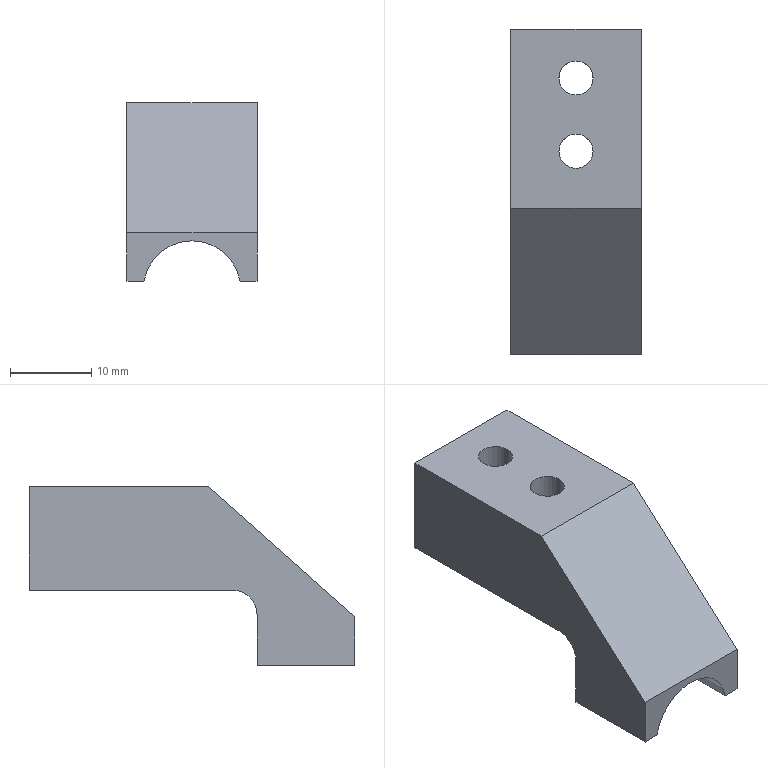Component | SolidWorks | CCDBlankingGripper-6 | 1 solid | 20 faces | box 16 x 40 x 22 mm | volume 5501 mm3 | plane 14 | cylinder 6 | commonest cylinder face diameters 4.2 x4 12 x1 6 x1 | material Q235
STEP:
#1=COLOUR_RGB('',0.7922,0.8196,0.9333);
#2=FILL_AREA_STYLE_COLOUR('',#1);
#3=FILL_AREA_STYLE('',(#2));
#4=SURFACE_STYLE_FILL_AREA(#3);
#5=SURFACE_SIDE_STYLE('',(#4));
#6=SURFACE_STYLE_USAGE(.BOTH.,#5);
#7=PRESENTATION_STYLE_ASSIGNMENT((#6));
#8=CARTESIAN_POINT('',(-6.173,11.207,-4.186));
#9=VERTEX_POINT('',#8);
#10=CARTESIAN_POINT('',(-6.339,11.207,-4.186));
#11=VERTEX_POINT('',#10);
#12=CARTESIAN_POINT('',(-6.256,11.207,-4.186));
#13=DIRECTION('',(-0.,0.,-1.));
#14=DIRECTION('',(0.,-1.,0.));
#15=AXIS2_PLACEMENT_3D('',#12,#13,#14);
#16=CIRCLE('',#15,0.08268);
#17=EDGE_CURVE('',#9,#11,#16,.T.);
#18=ORIENTED_EDGE('',*,*,#17,.T.);
#19=CARTESIAN_POINT('',(-6.339,11.207,-3.92));
#20=VERTEX_POINT('',#19);
#21=CARTESIAN_POINT('',(-6.339,11.207,-3.92));
#22=DIRECTION('',(0.,-0.,1.));
#23=VECTOR('',#22,39.37);
#24=LINE('',#21,#23);
#25=EDGE_CURVE('',#11,#20,#24,.T.);
#26=ORIENTED_EDGE('',*,*,#25,.T.);
#27=CARTESIAN_POINT('',(-6.173,11.207,-3.92));
#28=VERTEX_POINT('',#27);
#29=CARTESIAN_POINT('',(-6.256,11.207,-3.92));
#30=DIRECTION('',(0.,-0.,1.));
#31=DIRECTION('',(1.,0.,0.));
#32=AXIS2_PLACEMENT_3D('',#29,#30,#31);
#33=CIRCLE('',#32,0.08268);
#34=EDGE_CURVE('',#20,#28,#33,.T.);
#35=ORIENTED_EDGE('',*,*,#34,.T.);
#36=CARTESIAN_POINT('',(-6.173,11.207,-3.92));
#37=DIRECTION('',(0.,-0.,1.));
#38=VECTOR('',#37,39.37);
#39=LINE('',#36,#38);
#40=EDGE_CURVE('',#9,#28,#39,.T.);
#41=ORIENTED_EDGE('',*,*,#40,.F.);
#42=EDGE_LOOP('',(#18,#26,#35,#41));
#43=FACE_OUTER_BOUND('',#42,.T.);
#44=CARTESIAN_POINT('',(-6.256,11.207,-3.92));
#45=DIRECTION('',(0.,-0.,1.));
#46=DIRECTION('',(1.,0.,0.));
#47=AXIS2_PLACEMENT_3D('',#44,#45,#46);
#48=CYLINDRICAL_SURFACE('',#47,0.08268);
#49=ADVANCED_FACE('',(#43),#48,.F.);
#50=CARTESIAN_POINT('',(-6.173,10.853,-4.186));
#51=VERTEX_POINT('',#50);
#52=CARTESIAN_POINT('',(-6.339,10.853,-4.186));
#53=VERTEX_POINT('',#52);
#54=CARTESIAN_POINT('',(-6.256,10.853,-4.186));
#55=DIRECTION('',(-0.,0.,-1.));
#56=DIRECTION('',(0.,-1.,0.));
#57=AXIS2_PLACEMENT_3D('',#54,#55,#56);
#58=CIRCLE('',#57,0.08268);
#59=EDGE_CURVE('',#51,#53,#58,.T.);
#60=ORIENTED_EDGE('',*,*,#59,.T.);
#61=CARTESIAN_POINT('',(-6.339,10.853,-3.92));
#62=VERTEX_POINT('',#61);
#63=CARTESIAN_POINT('',(-6.339,10.853,-3.92));
#64=DIRECTION('',(0.,-0.,1.));
#65=VECTOR('',#64,39.37);
#66=LINE('',#63,#65);
#67=EDGE_CURVE('',#53,#62,#66,.T.);
#68=ORIENTED_EDGE('',*,*,#67,.T.);
#69=CARTESIAN_POINT('',(-6.173,10.853,-3.92));
#70=VERTEX_POINT('',#69);
#71=CARTESIAN_POINT('',(-6.256,10.853,-3.92));
#72=DIRECTION('',(0.,-0.,1.));
#73=DIRECTION('',(1.,0.,0.));
#74=AXIS2_PLACEMENT_3D('',#71,#72,#73);
#75=CIRCLE('',#74,0.08268);
#76=EDGE_CURVE('',#62,#70,#75,.T.);
#77=ORIENTED_EDGE('',*,*,#76,.T.);
#78=CARTESIAN_POINT('',(-6.173,10.853,-3.92));
#79=DIRECTION('',(0.,-0.,1.));
#80=VECTOR('',#79,39.37);
#81=LINE('',#78,#80);
#82=EDGE_CURVE('',#51,#70,#81,.T.);
#83=ORIENTED_EDGE('',*,*,#82,.F.);
#84=EDGE_LOOP('',(#60,#68,#77,#83));
#85=FACE_OUTER_BOUND('',#84,.T.);
#86=CARTESIAN_POINT('',(-6.256,10.853,-3.92));
#87=DIRECTION('',(0.,-0.,1.));
#88=DIRECTION('',(1.,0.,0.));
#89=AXIS2_PLACEMENT_3D('',#86,#87,#88);
#90=CYLINDRICAL_SURFACE('',#89,0.08268);
#91=ADVANCED_FACE('',(#85),#90,.F.);
#92=CARTESIAN_POINT('',(-6.571,10.341,-4.786));
#93=VERTEX_POINT('',#92);
#94=CARTESIAN_POINT('',(-6.489,10.341,-4.786));
#95=VERTEX_POINT('',#94);
#96=CARTESIAN_POINT('',(-5.941,10.341,-4.786));
#97=DIRECTION('',(1.,-0.,-0.));
#98=VECTOR('',#97,39.37);
#99=LINE('',#96,#98);
#100=EDGE_CURVE('',#93,#95,#99,.T.);
#101=ORIENTED_EDGE('',*,*,#100,.T.);
#102=CARTESIAN_POINT('',(-6.489,9.869,-4.786));
#103=VERTEX_POINT('',#102);
#104=CARTESIAN_POINT('',(-6.489,11.443,-4.786));
#105=DIRECTION('',(-0.,-1.,-0.));
#106=VECTOR('',#105,39.37);
#107=LINE('',#104,#106);
#108=EDGE_CURVE('',#95,#103,#107,.T.);
#109=ORIENTED_EDGE('',*,*,#108,.T.);
#110=CARTESIAN_POINT('',(-6.571,9.869,-4.786));
#111=VERTEX_POINT('',#110);
#112=CARTESIAN_POINT('',(-5.941,9.869,-4.786));
#113=DIRECTION('',(-1.,0.,0.));
#114=VECTOR('',#113,39.37);
#115=LINE('',#112,#114);
#116=EDGE_CURVE('',#103,#111,#115,.T.);
#117=ORIENTED_EDGE('',*,*,#116,.T.);
#118=CARTESIAN_POINT('',(-6.571,9.869,-4.786));
#119=DIRECTION('',(0.,1.,0.));
#120=VECTOR('',#119,39.37);
#121=LINE('',#118,#120);
#122=EDGE_CURVE('',#111,#93,#121,.T.);
#123=ORIENTED_EDGE('',*,*,#122,.T.);
#124=EDGE_LOOP('',(#101,#109,#117,#123));
#125=FACE_OUTER_BOUND('',#124,.T.);
#126=CARTESIAN_POINT('',(-5.941,9.869,-4.786));
#127=DIRECTION('',(0.,-0.,1.));
#128=DIRECTION('',(1.,-0.,-0.));
#129=AXIS2_PLACEMENT_3D('',#126,#127,#128);
#130=PLANE('',#129);
#131=ADVANCED_FACE('',(#125),#130,.F.);
#132=ORIENTED_EDGE('',*,*,#116,.F.);
#133=CARTESIAN_POINT('',(-6.023,9.869,-4.786));
#134=VERTEX_POINT('',#133);
#135=CARTESIAN_POINT('',(-6.256,9.869,-4.826));
#136=DIRECTION('',(-0.,-1.,-0.));
#137=DIRECTION('',(1.,-0.,0.));
#138=AXIS2_PLACEMENT_3D('',#135,#136,#137);
#139=CIRCLE('',#138,0.2362);
#140=EDGE_CURVE('',#134,#103,#139,.T.);
#141=ORIENTED_EDGE('',*,*,#140,.F.);
#142=CARTESIAN_POINT('',(-5.941,9.869,-4.786));
#143=VERTEX_POINT('',#142);
#144=CARTESIAN_POINT('',(-5.941,9.869,-4.786));
#145=DIRECTION('',(-1.,0.,0.));
#146=VECTOR('',#145,39.37);
#147=LINE('',#144,#146);
#148=EDGE_CURVE('',#143,#134,#147,.T.);
#149=ORIENTED_EDGE('',*,*,#148,.F.);
#150=CARTESIAN_POINT('',(-5.941,9.869,-4.55));
#151=VERTEX_POINT('',#150);
#152=CARTESIAN_POINT('',(-5.941,9.869,-4.786));
#153=DIRECTION('',(-0.,0.,-1.));
#154=VECTOR('',#153,39.37);
#155=LINE('',#152,#154);
#156=EDGE_CURVE('',#151,#143,#155,.T.);
#157=ORIENTED_EDGE('',*,*,#156,.F.);
#158=CARTESIAN_POINT('',(-6.571,9.869,-4.55));
#159=VERTEX_POINT('',#158);
#160=CARTESIAN_POINT('',(-6.571,9.869,-4.55));
#161=DIRECTION('',(1.,-0.,-0.));
#162=VECTOR('',#161,39.37);
#163=LINE('',#160,#162);
#164=EDGE_CURVE('',#159,#151,#163,.T.);
#165=ORIENTED_EDGE('',*,*,#164,.F.);
#166=CARTESIAN_POINT('',(-6.571,9.869,-4.786));
#167=DIRECTION('',(-0.,0.,-1.));
#168=VECTOR('',#167,39.37);
#169=LINE('',#166,#168);
#170=EDGE_CURVE('',#159,#111,#169,.T.);
#171=ORIENTED_EDGE('',*,*,#170,.T.);
#172=EDGE_LOOP('',(#132,#141,#149,#157,#165,#171));
#173=FACE_OUTER_BOUND('',#172,.T.);
#174=CARTESIAN_POINT('',(-5.941,9.869,-4.786));
#175=DIRECTION('',(0.,1.,0.));
#176=DIRECTION('',(-1.,0.,0.));
#177=AXIS2_PLACEMENT_3D('',#174,#175,#176);
#178=PLANE('',#177);
#179=ADVANCED_FACE('',(#173),#178,.F.);
#180=ORIENTED_EDGE('',*,*,#148,.T.);
#181=CARTESIAN_POINT('',(-6.023,10.341,-4.786));
#182=VERTEX_POINT('',#181);
#183=CARTESIAN_POINT('',(-6.023,11.443,-4.786));
#184=DIRECTION('',(0.,1.,0.));
#185=VECTOR('',#184,39.37);
#186=LINE('',#183,#185);
#187=EDGE_CURVE('',#134,#182,#186,.T.);
#188=ORIENTED_EDGE('',*,*,#187,.T.);
#189=CARTESIAN_POINT('',(-5.941,10.341,-4.786));
#190=VERTEX_POINT('',#189);
#191=CARTESIAN_POINT('',(-5.941,10.341,-4.786));
#192=DIRECTION('',(1.,-0.,-0.));
#193=VECTOR('',#192,39.37);
#194=LINE('',#191,#193);
#195=EDGE_CURVE('',#182,#190,#194,.T.);
#196=ORIENTED_EDGE('',*,*,#195,.T.);
#197=CARTESIAN_POINT('',(-5.941,9.869,-4.786));
#198=DIRECTION('',(0.,1.,0.));
#199=VECTOR('',#198,39.37);
#200=LINE('',#197,#199);
#201=EDGE_CURVE('',#143,#190,#200,.T.);
#202=ORIENTED_EDGE('',*,*,#201,.F.);
#203=EDGE_LOOP('',(#180,#188,#196,#202));
#204=FACE_OUTER_BOUND('',#203,.T.);
#205=CARTESIAN_POINT('',(-5.941,9.869,-4.786));
#206=DIRECTION('',(0.,-0.,1.));
#207=DIRECTION('',(1.,-0.,-0.));
#208=AXIS2_PLACEMENT_3D('',#205,#206,#207);
#209=PLANE('',#208);
#210=ADVANCED_FACE('',(#204),#209,.F.);
#211=CARTESIAN_POINT('',(-6.02,11.443,-4.186));
#212=VERTEX_POINT('',#211);
#213=CARTESIAN_POINT('',(-6.492,11.443,-4.186));
#214=VERTEX_POINT('',#213);
#215=CARTESIAN_POINT('',(-5.941,11.443,-4.186));
#216=DIRECTION('',(-1.,0.,0.));
#217=VECTOR('',#216,39.37);
#218=LINE('',#215,#217);
#219=EDGE_CURVE('',#212,#214,#218,.T.);
#220=ORIENTED_EDGE('',*,*,#219,.T.);
#221=CARTESIAN_POINT('',(-6.492,11.443,-4.422));
#222=VERTEX_POINT('',#221);
#223=CARTESIAN_POINT('',(-6.492,11.443,-4.786));
#224=DIRECTION('',(-0.,0.,-1.));
#225=VECTOR('',#224,39.37);
#226=LINE('',#223,#225);
#227=EDGE_CURVE('',#214,#222,#226,.T.);
#228=ORIENTED_EDGE('',*,*,#227,.T.);
#229=CARTESIAN_POINT('',(-6.571,11.443,-4.422));
#230=VERTEX_POINT('',#229);
#231=CARTESIAN_POINT('',(-6.571,11.443,-4.422));
#232=DIRECTION('',(1.,-0.,-0.));
#233=VECTOR('',#232,39.37);
#234=LINE('',#231,#233);
#235=EDGE_CURVE('',#230,#222,#234,.T.);
#236=ORIENTED_EDGE('',*,*,#235,.F.);
#237=CARTESIAN_POINT('',(-6.571,11.443,-3.92));
#238=VERTEX_POINT('',#237);
#239=CARTESIAN_POINT('',(-6.571,11.443,-4.786));
#240=DIRECTION('',(0.,-0.,1.));
#241=VECTOR('',#240,39.37);
#242=LINE('',#239,#241);
#243=EDGE_CURVE('',#230,#238,#242,.T.);
#244=ORIENTED_EDGE('',*,*,#243,.T.);
#245=CARTESIAN_POINT('',(-5.941,11.443,-3.92));
#246=VERTEX_POINT('',#245);
#247=CARTESIAN_POINT('',(-5.941,11.443,-3.92));
#248=DIRECTION('',(-1.,0.,0.));
#249=VECTOR('',#248,39.37);
#250=LINE('',#247,#249);
#251=EDGE_CURVE('',#246,#238,#250,.T.);
#252=ORIENTED_EDGE('',*,*,#251,.F.);
#253=CARTESIAN_POINT('',(-5.941,11.443,-4.422));
#254=VERTEX_POINT('',#253);
#255=CARTESIAN_POINT('',(-5.941,11.443,-4.786));
#256=DIRECTION('',(0.,-0.,1.));
#257=VECTOR('',#256,39.37);
#258=LINE('',#255,#257);
#259=EDGE_CURVE('',#254,#246,#258,.T.);
#260=ORIENTED_EDGE('',*,*,#259,.F.);
#261=CARTESIAN_POINT('',(-6.02,11.443,-4.422));
#262=VERTEX_POINT('',#261);
#263=CARTESIAN_POINT('',(-6.571,11.443,-4.422));
#264=DIRECTION('',(1.,-0.,-0.));
#265=VECTOR('',#264,39.37);
#266=LINE('',#263,#265);
#267=EDGE_CURVE('',#262,#254,#266,.T.);
#268=ORIENTED_EDGE('',*,*,#267,.F.);
#269=CARTESIAN_POINT('',(-6.02,11.443,-4.786));
#270=DIRECTION('',(0.,-0.,1.));
#271=VECTOR('',#270,39.37);
#272=LINE('',#269,#271);
#273=EDGE_CURVE('',#262,#212,#272,.T.);
#274=ORIENTED_EDGE('',*,*,#273,.T.);
#275=EDGE_LOOP('',(#220,#228,#236,#244,#252,#260,#268,#274));
#276=FACE_OUTER_BOUND('',#275,.T.);
#277=CARTESIAN_POINT('',(-5.941,11.443,-4.786));
#278=DIRECTION('',(-0.,-1.,-0.));
#279=DIRECTION('',(1.,-0.,-0.));
#280=AXIS2_PLACEMENT_3D('',#277,#278,#279);
#281=PLANE('',#280);
#282=ADVANCED_FACE('',(#276),#281,.F.);
#283=CARTESIAN_POINT('',(-6.256,11.207,-3.92));
#284=DIRECTION('',(0.,-0.,1.));
#285=DIRECTION('',(1.,0.,0.));
#286=AXIS2_PLACEMENT_3D('',#283,#284,#285);
#287=CIRCLE('',#286,0.08268);
#288=EDGE_CURVE('',#28,#20,#287,.T.);
#289=ORIENTED_EDGE('',*,*,#288,.F.);
#290=ORIENTED_EDGE('',*,*,#34,.F.);
#291=EDGE_LOOP('',(#289,#290));
#292=FACE_BOUND('',#291,.T.);
#293=CARTESIAN_POINT('',(-6.256,10.853,-3.92));
#294=DIRECTION('',(0.,-0.,1.));
#295=DIRECTION('',(1.,0.,0.));
#296=AXIS2_PLACEMENT_3D('',#293,#294,#295);
#297=CIRCLE('',#296,0.08268);
#298=EDGE_CURVE('',#70,#62,#297,.T.);
#299=ORIENTED_EDGE('',*,*,#298,.F.);
#300=ORIENTED_EDGE('',*,*,#76,.F.);
#301=EDGE_LOOP('',(#299,#300));
#302=FACE_BOUND('',#301,.T.);
#303=CARTESIAN_POINT('',(-6.571,10.577,-3.92));
#304=VERTEX_POINT('',#303);
#305=CARTESIAN_POINT('',(-6.571,9.869,-3.92));
#306=DIRECTION('',(-0.,-1.,-0.));
#307=VECTOR('',#306,39.37);
#308=LINE('',#305,#307);
#309=EDGE_CURVE('',#238,#304,#308,.T.);
#310=ORIENTED_EDGE('',*,*,#309,.T.);
#311=CARTESIAN_POINT('',(-5.941,10.577,-3.92));
#312=VERTEX_POINT('',#311);
#313=CARTESIAN_POINT('',(-6.571,10.577,-3.92));
#314=DIRECTION('',(1.,-0.,-0.));
#315=VECTOR('',#314,39.37);
#316=LINE('',#313,#315);
#317=EDGE_CURVE('',#304,#312,#316,.T.);
#318=ORIENTED_EDGE('',*,*,#317,.T.);
#319=CARTESIAN_POINT('',(-5.941,9.869,-3.92));
#320=DIRECTION('',(-0.,-1.,-0.));
#321=VECTOR('',#320,39.37);
#322=LINE('',#319,#321);
#323=EDGE_CURVE('',#246,#312,#322,.T.);
#324=ORIENTED_EDGE('',*,*,#323,.F.);
#325=ORIENTED_EDGE('',*,*,#251,.T.);
#326=EDGE_LOOP('',(#310,#318,#324,#325));
#327=FACE_OUTER_BOUND('',#326,.T.);
#328=CARTESIAN_POINT('',(-5.941,9.869,-3.92));
#329=DIRECTION('',(-0.,0.,-1.));
#330=DIRECTION('',(-1.,0.,0.));
#331=AXIS2_PLACEMENT_3D('',#328,#329,#330);
#332=PLANE('',#331);
#333=ADVANCED_FACE('',(#292,#302,#327),#332,.F.);
#334=ORIENTED_EDGE('',*,*,#201,.T.);
#335=CARTESIAN_POINT('',(-5.941,10.341,-4.54));
#336=VERTEX_POINT('',#335);
#337=CARTESIAN_POINT('',(-5.941,10.341,-4.422));
#338=DIRECTION('',(-0.,0.,-1.));
#339=VECTOR('',#338,39.37);
#340=LINE('',#337,#339);
#341=EDGE_CURVE('',#336,#190,#340,.T.);
#342=ORIENTED_EDGE('',*,*,#341,.F.);
#343=CARTESIAN_POINT('',(-5.941,10.459,-4.422));
#344=VERTEX_POINT('',#343);
#345=CARTESIAN_POINT('',(-5.941,10.459,-4.54));
#346=DIRECTION('',(-1.,0.,0.));
#347=DIRECTION('',(-0.,-1.,0.));
#348=AXIS2_PLACEMENT_3D('',#345,#346,#347);
#349=CIRCLE('',#348,0.1181);
#350=EDGE_CURVE('',#336,#344,#349,.T.);
#351=ORIENTED_EDGE('',*,*,#350,.T.);
#352=CARTESIAN_POINT('',(-5.941,11.443,-4.422));
#353=DIRECTION('',(-0.,-1.,-0.));
#354=VECTOR('',#353,39.37);
#355=LINE('',#352,#354);
#356=EDGE_CURVE('',#254,#344,#355,.T.);
#357=ORIENTED_EDGE('',*,*,#356,.F.);
#358=ORIENTED_EDGE('',*,*,#259,.T.);
#359=ORIENTED_EDGE('',*,*,#323,.T.);
#360=CARTESIAN_POINT('',(-5.941,9.869,-4.55));
#361=DIRECTION('',(0.,0.7474,0.6644));
#362=VECTOR('',#361,39.37);
#363=LINE('',#360,#362);
#364=EDGE_CURVE('',#151,#312,#363,.T.);
#365=ORIENTED_EDGE('',*,*,#364,.F.);
#366=ORIENTED_EDGE('',*,*,#156,.T.);
#367=EDGE_LOOP('',(#334,#342,#351,#357,#358,#359,#365,#366));
#368=FACE_OUTER_BOUND('',#367,.T.);
#369=CARTESIAN_POINT('',(-5.941,9.869,-4.786));
#370=DIRECTION('',(-1.,0.,0.));
#371=DIRECTION('',(-0.,-1.,-0.));
#372=AXIS2_PLACEMENT_3D('',#369,#370,#371);
#373=PLANE('',#372);
#374=ADVANCED_FACE('',(#368),#373,.F.);
#375=CARTESIAN_POINT('',(-6.571,10.459,-4.422));
#376=VERTEX_POINT('',#375);
#377=CARTESIAN_POINT('',(-6.571,11.443,-4.422));
#378=DIRECTION('',(-0.,-1.,-0.));
#379=VECTOR('',#378,39.37);
#380=LINE('',#377,#379);
#381=EDGE_CURVE('',#230,#376,#380,.T.);
#382=ORIENTED_EDGE('',*,*,#381,.T.);
#383=CARTESIAN_POINT('',(-6.571,10.341,-4.54));
#384=VERTEX_POINT('',#383);
#385=CARTESIAN_POINT('',(-6.571,10.459,-4.54));
#386=DIRECTION('',(1.,-0.,-0.));
#387=DIRECTION('',(-0.,-1.,0.));
#388=AXIS2_PLACEMENT_3D('',#385,#386,#387);
#389=CIRCLE('',#388,0.1181);
#390=EDGE_CURVE('',#376,#384,#389,.T.);
#391=ORIENTED_EDGE('',*,*,#390,.T.);
#392=CARTESIAN_POINT('',(-6.571,10.341,-4.422));
#393=DIRECTION('',(-0.,0.,-1.));
#394=VECTOR('',#393,39.37);
#395=LINE('',#392,#394);
#396=EDGE_CURVE('',#384,#93,#395,.T.);
#397=ORIENTED_EDGE('',*,*,#396,.T.);
#398=ORIENTED_EDGE('',*,*,#122,.F.);
#399=ORIENTED_EDGE('',*,*,#170,.F.);
#400=CARTESIAN_POINT('',(-6.571,9.869,-4.55));
#401=DIRECTION('',(0.,0.7474,0.6644));
#402=VECTOR('',#401,39.37);
#403=LINE('',#400,#402);
#404=EDGE_CURVE('',#159,#304,#403,.T.);
#405=ORIENTED_EDGE('',*,*,#404,.T.);
#406=ORIENTED_EDGE('',*,*,#309,.F.);
#407=ORIENTED_EDGE('',*,*,#243,.F.);
#408=EDGE_LOOP('',(#382,#391,#397,#398,#399,#405,#406,#407));
#409=FACE_OUTER_BOUND('',#408,.T.);
#410=CARTESIAN_POINT('',(-6.571,9.869,-4.786));
#411=DIRECTION('',(-1.,0.,0.));
#412=DIRECTION('',(-0.,-1.,-0.));
#413=AXIS2_PLACEMENT_3D('',#410,#411,#412);
#414=PLANE('',#413);
#415=ADVANCED_FACE('',(#409),#414,.T.);
#416=ORIENTED_EDGE('',*,*,#364,.T.);
#417=ORIENTED_EDGE('',*,*,#317,.F.);
#418=ORIENTED_EDGE('',*,*,#404,.F.);
#419=ORIENTED_EDGE('',*,*,#164,.T.);
#420=EDGE_LOOP('',(#416,#417,#418,#419));
#421=FACE_OUTER_BOUND('',#420,.T.);
#422=CARTESIAN_POINT('',(-6.571,9.869,-4.55));
#423=DIRECTION('',(0.,0.6644,-0.7474));
#424=DIRECTION('',(0.,0.7474,0.6644));
#425=AXIS2_PLACEMENT_3D('',#422,#423,#424);
#426=PLANE('',#425);
#427=ADVANCED_FACE('',(#421),#426,.F.);
#428=ORIENTED_EDGE('',*,*,#396,.F.);
#429=CARTESIAN_POINT('',(-5.941,10.341,-4.54));
#430=DIRECTION('',(1.,-0.,-0.));
#431=VECTOR('',#430,39.37);
#432=LINE('',#429,#431);
#433=EDGE_CURVE('',#384,#336,#432,.T.);
#434=ORIENTED_EDGE('',*,*,#433,.T.);
#435=ORIENTED_EDGE('',*,*,#341,.T.);
#436=ORIENTED_EDGE('',*,*,#195,.F.);
#437=CARTESIAN_POINT('',(-6.256,10.341,-4.826));
#438=DIRECTION('',(-0.,-1.,-0.));
#439=DIRECTION('',(0.,0.,-1.));
#440=AXIS2_PLACEMENT_3D('',#437,#438,#439);
#441=CIRCLE('',#440,0.2362);
#442=EDGE_CURVE('',#182,#95,#441,.T.);
#443=ORIENTED_EDGE('',*,*,#442,.T.);
#444=ORIENTED_EDGE('',*,*,#100,.F.);
#445=EDGE_LOOP('',(#428,#434,#435,#436,#443,#444));
#446=FACE_OUTER_BOUND('',#445,.T.);
#447=CARTESIAN_POINT('',(-6.571,10.341,-4.422));
#448=DIRECTION('',(-0.,-1.,-0.));
#449=DIRECTION('',(-0.,0.,-1.));
#450=AXIS2_PLACEMENT_3D('',#447,#448,#449);
#451=PLANE('',#450);
#452=ADVANCED_FACE('',(#446),#451,.F.);
#453=ORIENTED_EDGE('',*,*,#356,.T.);
#454=CARTESIAN_POINT('',(-6.571,10.459,-4.422));
#455=DIRECTION('',(-1.,0.,0.));
#456=VECTOR('',#455,39.37);
#457=LINE('',#454,#456);
#458=EDGE_CURVE('',#344,#376,#457,.T.);
#459=ORIENTED_EDGE('',*,*,#458,.T.);
#460=ORIENTED_EDGE('',*,*,#381,.F.);
#461=ORIENTED_EDGE('',*,*,#235,.T.);
#462=CARTESIAN_POINT('',(-6.492,10.656,-4.422));
#463=VERTEX_POINT('',#462);
#464=CARTESIAN_POINT('',(-6.492,11.54,-4.422));
#465=DIRECTION('',(0.,1.,0.));
#466=VECTOR('',#465,39.37);
#467=LINE('',#464,#466);
#468=EDGE_CURVE('',#463,#222,#467,.T.);
#469=ORIENTED_EDGE('',*,*,#468,.F.);
#470=CARTESIAN_POINT('',(-6.02,10.656,-4.422));
#471=VERTEX_POINT('',#470);
#472=CARTESIAN_POINT('',(-6.02,10.656,-4.422));
#473=DIRECTION('',(-1.,0.,0.));
#474=VECTOR('',#473,39.37);
#475=LINE('',#472,#474);
#476=EDGE_CURVE('',#471,#463,#475,.T.);
#477=ORIENTED_EDGE('',*,*,#476,.F.);
#478=CARTESIAN_POINT('',(-6.02,11.54,-4.422));
#479=DIRECTION('',(-0.,-1.,-0.));
#480=VECTOR('',#479,39.37);
#481=LINE('',#478,#480);
#482=EDGE_CURVE('',#262,#471,#481,.T.);
#483=ORIENTED_EDGE('',*,*,#482,.F.);
#484=ORIENTED_EDGE('',*,*,#267,.T.);
#485=EDGE_LOOP('',(#453,#459,#460,#461,#469,#477,#483,#484));
#486=FACE_OUTER_BOUND('',#485,.T.);
#487=CARTESIAN_POINT('',(-6.571,11.443,-4.422));
#488=DIRECTION('',(0.,-0.,1.));
#489=DIRECTION('',(-0.,-1.,-0.));
#490=AXIS2_PLACEMENT_3D('',#487,#488,#489);
#491=PLANE('',#490);
#492=ADVANCED_FACE('',(#486),#491,.F.);
#493=ORIENTED_EDGE('',*,*,#67,.F.);
#494=CARTESIAN_POINT('',(-6.256,10.853,-4.186));
#495=DIRECTION('',(-0.,0.,-1.));
#496=DIRECTION('',(0.,-1.,0.));
#497=AXIS2_PLACEMENT_3D('',#494,#495,#496);
#498=CIRCLE('',#497,0.08268);
#499=EDGE_CURVE('',#53,#51,#498,.T.);
#500=ORIENTED_EDGE('',*,*,#499,.T.);
#501=ORIENTED_EDGE('',*,*,#82,.T.);
#502=ORIENTED_EDGE('',*,*,#298,.T.);
#503=EDGE_LOOP('',(#493,#500,#501,#502));
#504=FACE_OUTER_BOUND('',#503,.T.);
#505=CARTESIAN_POINT('',(-6.256,10.853,-3.92));
#506=DIRECTION('',(0.,-0.,1.));
#507=DIRECTION('',(1.,0.,0.));
#508=AXIS2_PLACEMENT_3D('',#505,#506,#507);
#509=CYLINDRICAL_SURFACE('',#508,0.08268);
#510=ADVANCED_FACE('',(#504),#509,.F.);
#511=ORIENTED_EDGE('',*,*,#25,.F.);
#512=CARTESIAN_POINT('',(-6.256,11.207,-4.186));
#513=DIRECTION('',(-0.,0.,-1.));
#514=DIRECTION('',(0.,-1.,0.));
#515=AXIS2_PLACEMENT_3D('',#512,#513,#514);
#516=CIRCLE('',#515,0.08268);
#517=EDGE_CURVE('',#11,#9,#516,.T.);
#518=ORIENTED_EDGE('',*,*,#517,.T.);
#519=ORIENTED_EDGE('',*,*,#40,.T.);
#520=ORIENTED_EDGE('',*,*,#288,.T.);
#521=EDGE_LOOP('',(#511,#518,#519,#520));
#522=FACE_OUTER_BOUND('',#521,.T.);
#523=CARTESIAN_POINT('',(-6.256,11.207,-3.92));
#524=DIRECTION('',(0.,-0.,1.));
#525=DIRECTION('',(1.,0.,0.));
#526=AXIS2_PLACEMENT_3D('',#523,#524,#525);
#527=CYLINDRICAL_SURFACE('',#526,0.08268);
#528=ADVANCED_FACE('',(#522),#527,.F.);
#529=CARTESIAN_POINT('',(-6.492,10.656,-4.186));
#530=VERTEX_POINT('',#529);
#531=CARTESIAN_POINT('',(-6.492,11.54,-4.186));
#532=DIRECTION('',(0.,1.,0.));
#533=VECTOR('',#532,39.37);
#534=LINE('',#531,#533);
#535=EDGE_CURVE('',#530,#214,#534,.T.);
#536=ORIENTED_EDGE('',*,*,#535,.F.);
#537=CARTESIAN_POINT('',(-6.492,10.656,-4.186));
#538=DIRECTION('',(-0.,0.,-1.));
#539=VECTOR('',#538,39.37);
#540=LINE('',#537,#539);
#541=EDGE_CURVE('',#530,#463,#540,.T.);
#542=ORIENTED_EDGE('',*,*,#541,.T.);
#543=ORIENTED_EDGE('',*,*,#468,.T.);
#544=ORIENTED_EDGE('',*,*,#227,.F.);
#545=EDGE_LOOP('',(#536,#542,#543,#544));
#546=FACE_OUTER_BOUND('',#545,.T.);
#547=CARTESIAN_POINT('',(-6.492,11.54,-4.186));
#548=DIRECTION('',(-1.,0.,0.));
#549=DIRECTION('',(-0.,-1.,-0.));
#550=AXIS2_PLACEMENT_3D('',#547,#548,#549);
#551=PLANE('',#550);
#552=ADVANCED_FACE('',(#546),#551,.F.);
#553=ORIENTED_EDGE('',*,*,#482,.T.);
#554=CARTESIAN_POINT('',(-6.02,10.656,-4.186));
#555=VERTEX_POINT('',#554);
#556=CARTESIAN_POINT('',(-6.02,10.656,-4.186));
#557=DIRECTION('',(-0.,0.,-1.));
#558=VECTOR('',#557,39.37);
#559=LINE('',#556,#558);
#560=EDGE_CURVE('',#555,#471,#559,.T.);
#561=ORIENTED_EDGE('',*,*,#560,.F.);
#562=CARTESIAN_POINT('',(-6.02,11.54,-4.186));
#563=DIRECTION('',(-0.,-1.,-0.));
#564=VECTOR('',#563,39.37);
#565=LINE('',#562,#564);
#566=EDGE_CURVE('',#212,#555,#565,.T.);
#567=ORIENTED_EDGE('',*,*,#566,.F.);
#568=ORIENTED_EDGE('',*,*,#273,.F.);
#569=EDGE_LOOP('',(#553,#561,#567,#568));
#570=FACE_OUTER_BOUND('',#569,.T.);
#571=CARTESIAN_POINT('',(-6.02,11.54,-4.186));
#572=DIRECTION('',(1.,-0.,-0.));
#573=DIRECTION('',(0.,1.,0.));
#574=AXIS2_PLACEMENT_3D('',#571,#572,#573);
#575=PLANE('',#574);
#576=ADVANCED_FACE('',(#570),#575,.F.);
#577=ORIENTED_EDGE('',*,*,#17,.F.);
#578=ORIENTED_EDGE('',*,*,#517,.F.);
#579=EDGE_LOOP('',(#577,#578));
#580=FACE_BOUND('',#579,.T.);
#581=ORIENTED_EDGE('',*,*,#59,.F.);
#582=ORIENTED_EDGE('',*,*,#499,.F.);
#583=EDGE_LOOP('',(#581,#582));
#584=FACE_BOUND('',#583,.T.);
#585=ORIENTED_EDGE('',*,*,#566,.T.);
#586=CARTESIAN_POINT('',(-6.02,10.656,-4.186));
#587=DIRECTION('',(-1.,0.,0.));
#588=VECTOR('',#587,39.37);
#589=LINE('',#586,#588);
#590=EDGE_CURVE('',#555,#530,#589,.T.);
#591=ORIENTED_EDGE('',*,*,#590,.T.);
#592=ORIENTED_EDGE('',*,*,#535,.T.);
#593=ORIENTED_EDGE('',*,*,#219,.F.);
#594=EDGE_LOOP('',(#585,#591,#592,#593));
#595=FACE_OUTER_BOUND('',#594,.T.);
#596=CARTESIAN_POINT('',(-6.571,9.869,-4.186));
#597=DIRECTION('',(0.,-0.,1.));
#598=DIRECTION('',(-0.,-1.,-0.));
#599=AXIS2_PLACEMENT_3D('',#596,#597,#598);
#600=PLANE('',#599);
#601=ADVANCED_FACE('',(#580,#584,#595),#600,.F.);
#602=ORIENTED_EDGE('',*,*,#476,.T.);
#603=ORIENTED_EDGE('',*,*,#541,.F.);
#604=ORIENTED_EDGE('',*,*,#590,.F.);
#605=ORIENTED_EDGE('',*,*,#560,.T.);
#606=EDGE_LOOP('',(#602,#603,#604,#605));
#607=FACE_OUTER_BOUND('',#606,.T.);
#608=CARTESIAN_POINT('',(-6.02,10.656,-4.186));
#609=DIRECTION('',(-0.,-1.,-0.));
#610=DIRECTION('',(-0.,0.,-1.));
#611=AXIS2_PLACEMENT_3D('',#608,#609,#610);
#612=PLANE('',#611);
#613=ADVANCED_FACE('',(#607),#612,.F.);
#614=ORIENTED_EDGE('',*,*,#442,.F.);
#615=ORIENTED_EDGE('',*,*,#187,.F.);
#616=ORIENTED_EDGE('',*,*,#140,.T.);
#617=ORIENTED_EDGE('',*,*,#108,.F.);
#618=EDGE_LOOP('',(#614,#615,#616,#617));
#619=FACE_OUTER_BOUND('',#618,.T.);
#620=CARTESIAN_POINT('',(-6.256,11.443,-4.826));
#621=DIRECTION('',(-0.,-1.,-0.));
#622=DIRECTION('',(1.,-0.,0.));
#623=AXIS2_PLACEMENT_3D('',#620,#621,#622);
#624=CYLINDRICAL_SURFACE('',#623,0.2362);
#625=ADVANCED_FACE('',(#619),#624,.F.);
#626=ORIENTED_EDGE('',*,*,#390,.F.);
#627=ORIENTED_EDGE('',*,*,#458,.F.);
#628=ORIENTED_EDGE('',*,*,#350,.F.);
#629=ORIENTED_EDGE('',*,*,#433,.F.);
#630=EDGE_LOOP('',(#626,#627,#628,#629));
#631=FACE_OUTER_BOUND('',#630,.T.);
#632=CARTESIAN_POINT('',(-6.571,10.459,-4.54));
#633=DIRECTION('',(-1.,0.,0.));
#634=DIRECTION('',(-0.,-1.,0.));
#635=AXIS2_PLACEMENT_3D('',#632,#633,#634);
#636=CYLINDRICAL_SURFACE('',#635,0.1181);
#637=ADVANCED_FACE('',(#631),#636,.F.);
#638=CLOSED_SHELL('',(#49,#91,#131,#179,#210,#282,#333,#374,#415,#427,#452,#492,#510,#528,#552,#576,#601,#613,#625,#637));
#639=MANIFOLD_SOLID_BREP('',#638);
#640=STYLED_ITEM('',(#7),#639);
#641=PRESENTATION_LAYER_ASSIGNMENT('','',(#640));
#642=(LENGTH_UNIT()NAMED_UNIT(*)SI_UNIT($,.METRE.));
#643=LENGTH_MEASURE_WITH_UNIT(LENGTH_MEASURE(0.0254),#642);
#644=DIMENSIONAL_EXPONENTS(1.,0.,0.,0.,0.,0.,0.);
#645=(CONVERSION_BASED_UNIT('',#643)LENGTH_UNIT()NAMED_UNIT(#644));
#646=UNCERTAINTY_MEASURE_WITH_UNIT(LENGTH_MEASURE(0.00001),#645,'','');
#647=(NAMED_UNIT(*)PLANE_ANGLE_UNIT()SI_UNIT($,.RADIAN.));
#648=(NAMED_UNIT(*)SI_UNIT($,.STERADIAN.)SOLID_ANGLE_UNIT());
#649=(GEOMETRIC_REPRESENTATION_CONTEXT(3)GLOBAL_UNCERTAINTY_ASSIGNED_CONTEXT((#646))GLOBAL_UNIT_ASSIGNED_CONTEXT((#645,#647,#648))REPRESENTATION_CONTEXT('',''));
#650=MECHANICAL_DESIGN_GEOMETRIC_PRESENTATION_REPRESENTATION('',(#640),#649);
#651=CARTESIAN_POINT('',(0.,0.,0.));
#652=DIRECTION('',(0.,0.,1.));
#653=DIRECTION('',(1.,0.,0.));
#654=AXIS2_PLACEMENT_3D('',#651,#652,#653);
#655=(LENGTH_UNIT()NAMED_UNIT(*)SI_UNIT($,.METRE.));
#656=LENGTH_MEASURE_WITH_UNIT(LENGTH_MEASURE(0.0254),#655);
#657=DIMENSIONAL_EXPONENTS(1.,0.,0.,0.,0.,0.,0.);
#658=(CONVERSION_BASED_UNIT('',#656)LENGTH_UNIT()NAMED_UNIT(#657));
#659=UNCERTAINTY_MEASURE_WITH_UNIT(LENGTH_MEASURE(0.00001),#658,'','');
#660=(NAMED_UNIT(*)PLANE_ANGLE_UNIT()SI_UNIT($,.RADIAN.));
#661=(NAMED_UNIT(*)SI_UNIT($,.STERADIAN.)SOLID_ANGLE_UNIT());
#662=(GEOMETRIC_REPRESENTATION_CONTEXT(3)GLOBAL_UNCERTAINTY_ASSIGNED_CONTEXT((#659))GLOBAL_UNIT_ASSIGNED_CONTEXT((#658,#660,#661))REPRESENTATION_CONTEXT('',''));
#663=ADVANCED_BREP_SHAPE_REPRESENTATION('',(#639,#654),#662);